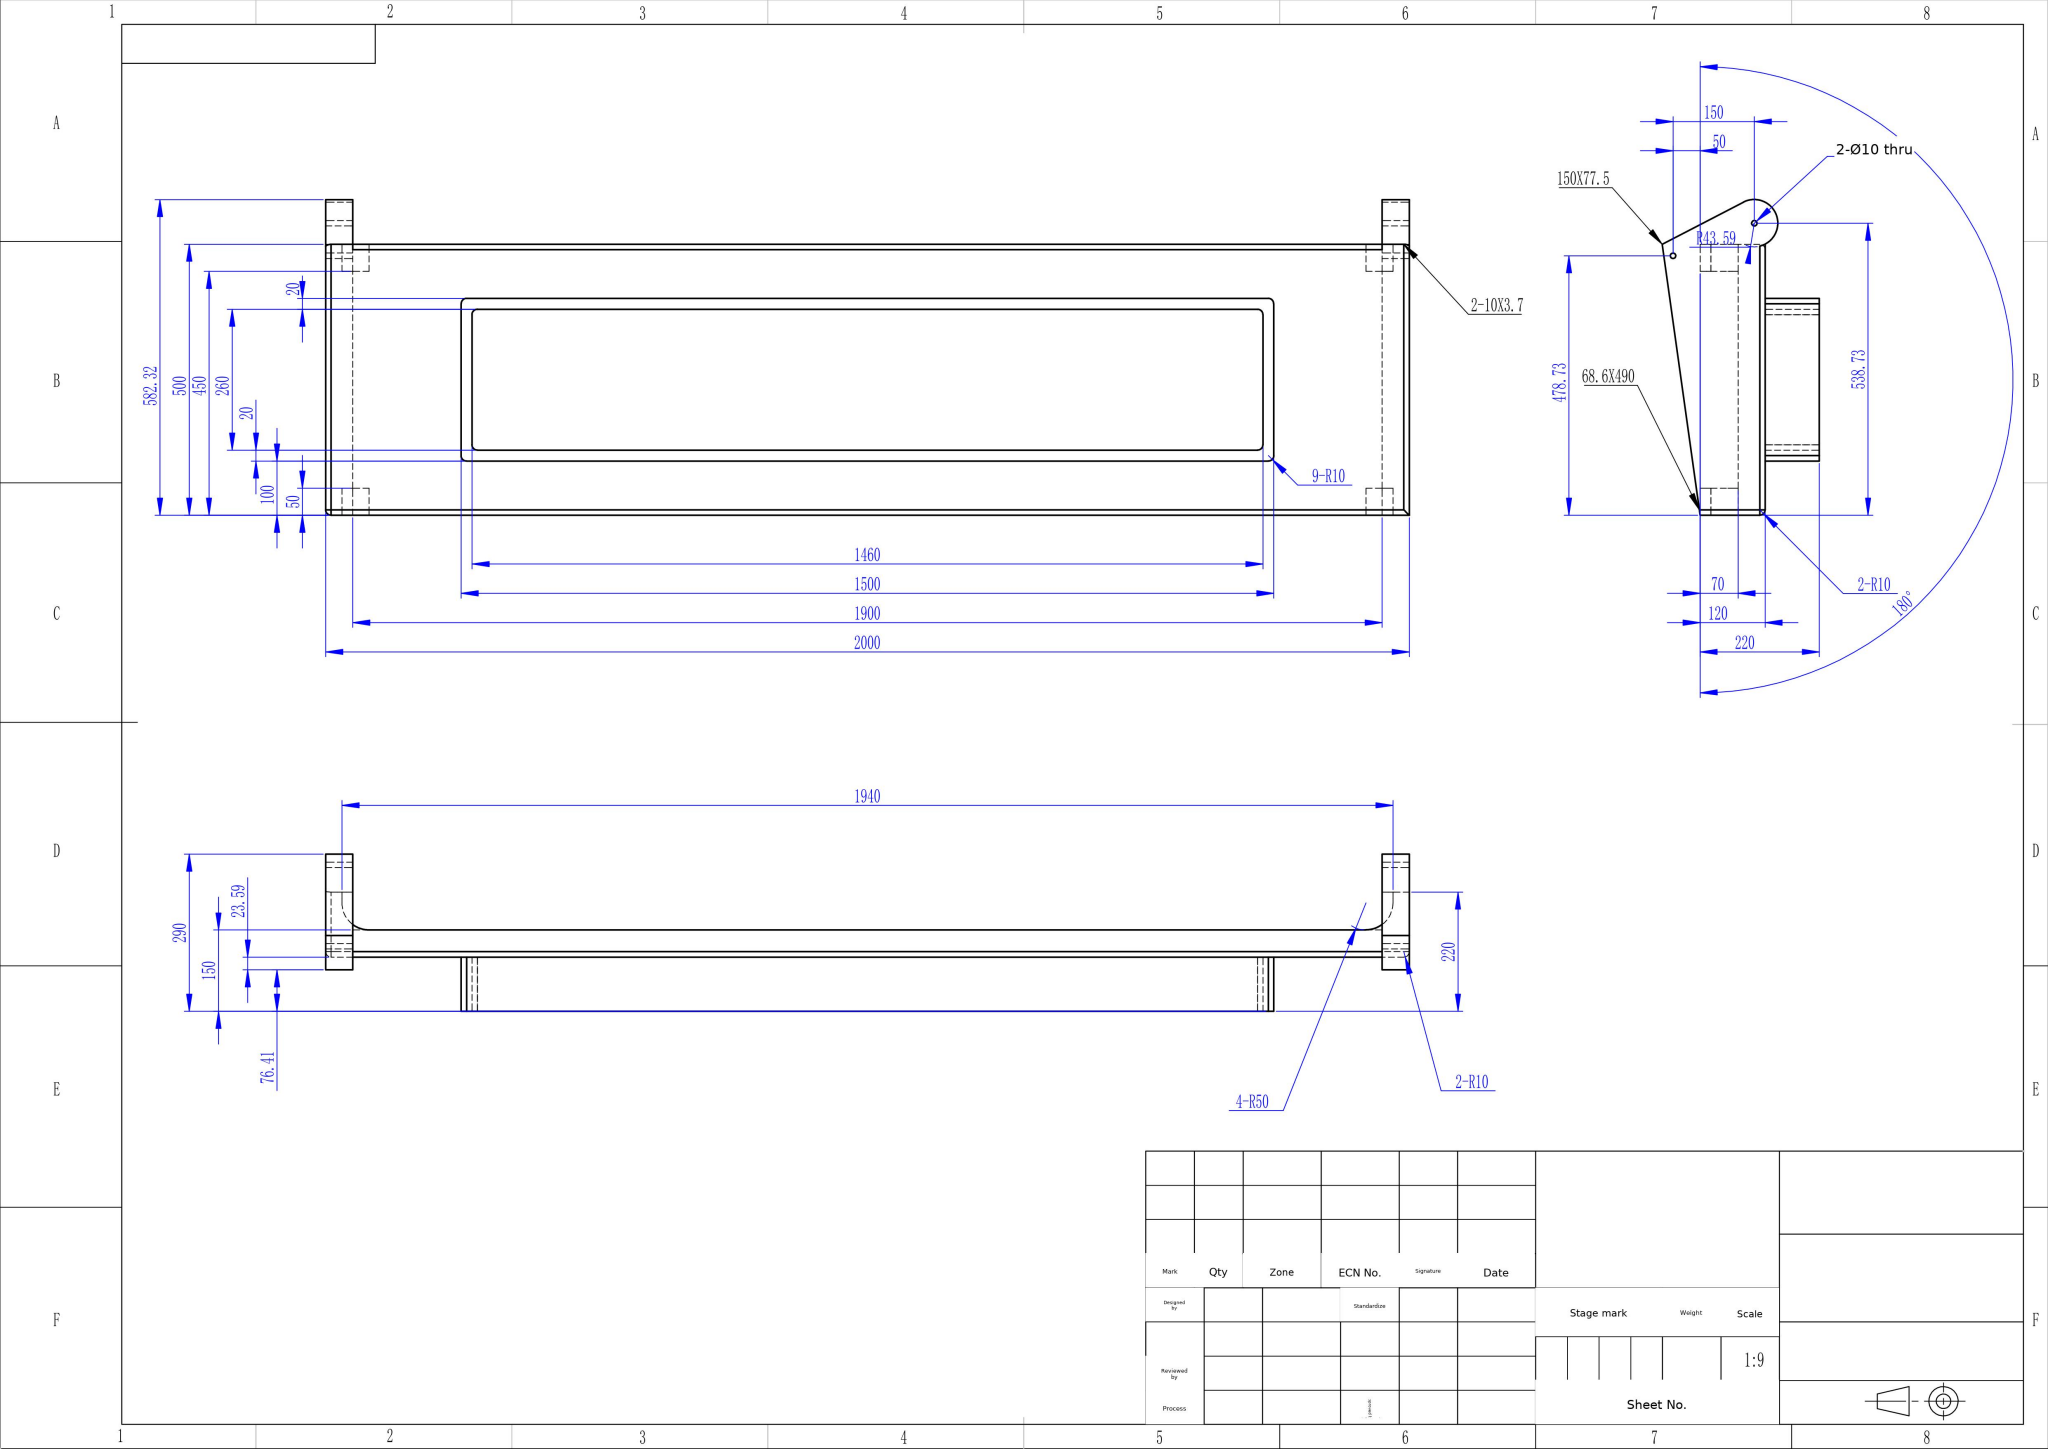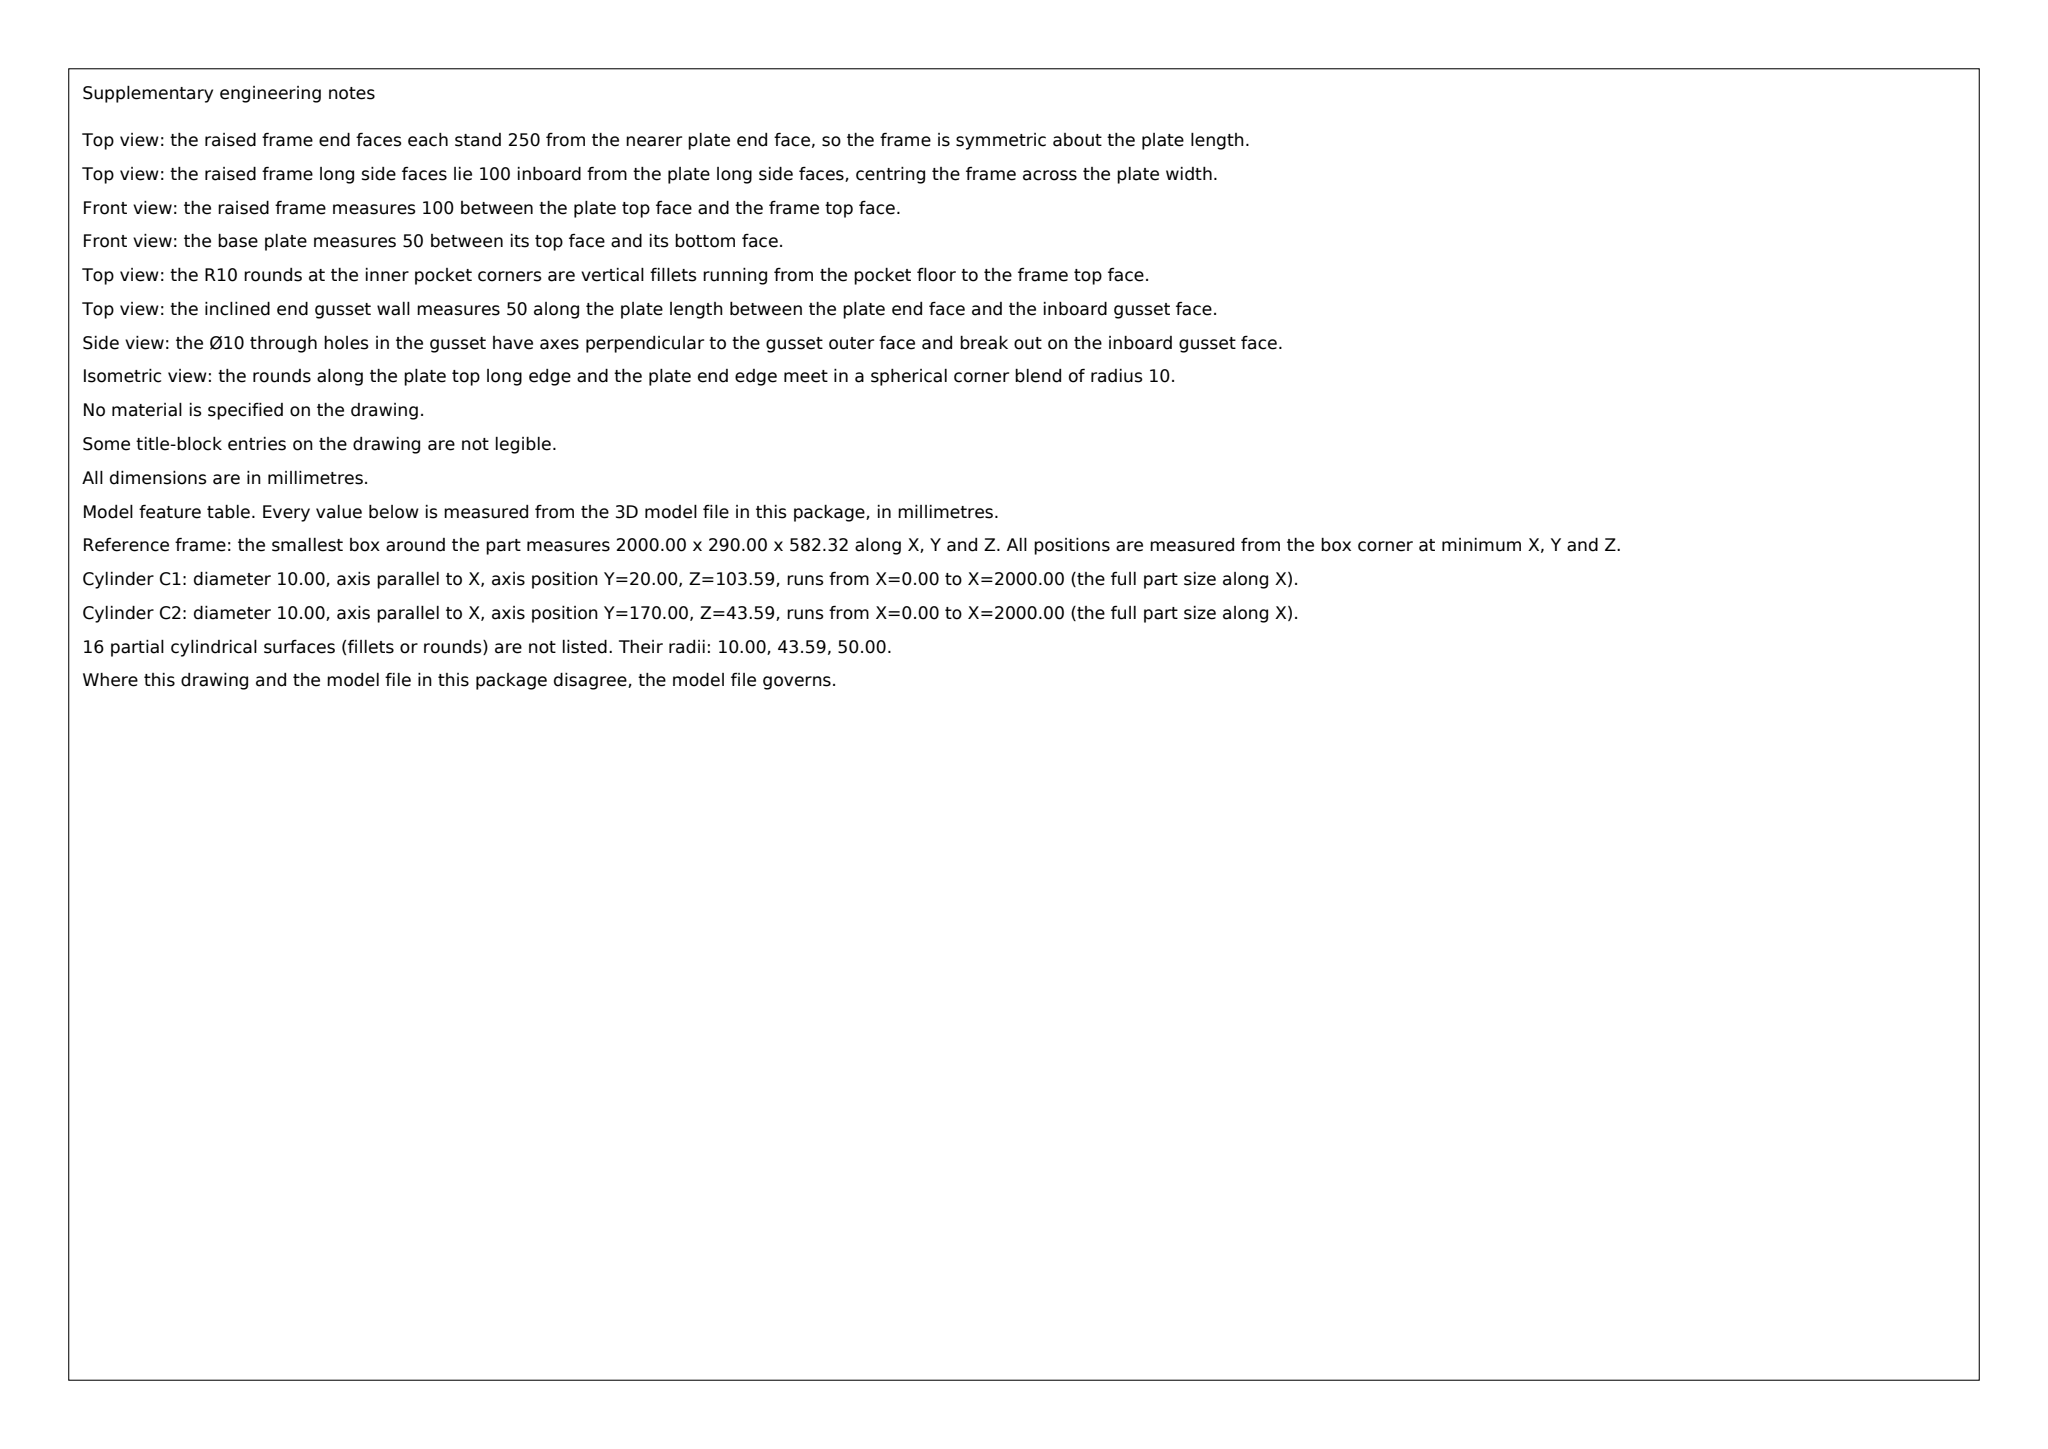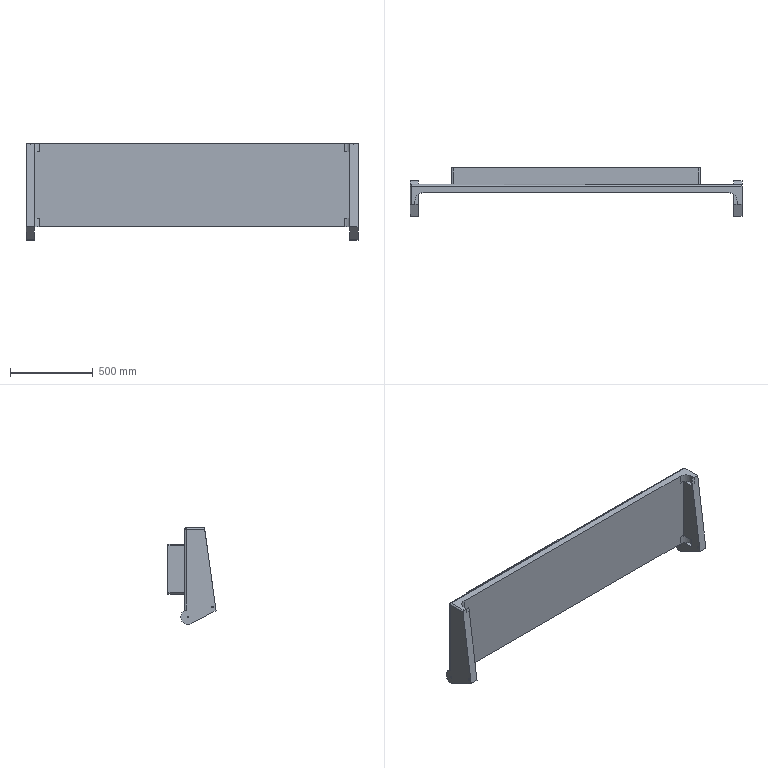Part | SolidWorks | mm | 1 solid | 69 faces | box 2000 x 290 x 582.32 mm | volume 63028481 mm3 | plane 40 | cylinder 28 | sphere 1 | commonest cylinder face diameters 20 x13 10 x8 100 x4 87.178 x3
Drawing notes:
2X Ø10 THRU END GUSSET, AXIS PARALLEL TO X, 50 DEEP FROM END FACE (X=0 AND X=2000); HOLE CENTERS AT Y=170, Z=43.59 AND Y=20, Z=103.59 FROM BBOX MIN CORNER. | from the solid: cylinders[dia,axis,pos,length]: [10.0,"x",[null,170.0,43.59],50.0] and [10.0,"x",[null,20.0,103.59],50.0]
GUSSET PLATE THICKNESS 50 ALONG X, FACES AT X=0/X=50 AND X=1950/X=2000 (SETS Ø10 HOLE AXIAL EXTENT). | from the solid: axis_planes[normal_axis,offset]: x=0.0, x=50.0, x=1950.0, x=2000.0
R43.59 ROUND END OF GUSSET IS CONCENTRIC WITH THE Ø10 HOLE AT Y=170, Z=43.59. | from the solid: cylinder [87.178,"x",[null,170.0,43.59],50.0] coincident with Ø10 hole at same y,z
ALL DIMENSIONS IN MILLIMETERS; OVERALL ENVELOPE 2000 X 290 X 582.32. | from the solid: bbox_xyz [2000.0, 290.0, 582.319] (mm)
build123d program:
from build123d import *

# Parameters (mm, degrees)
SKETCH1_W            = 2000
SKETCH1_H            = 500
BOSS_EXTRUDE1_DEPTH  = 50
BOSS_EXTRUDE2_DEPTH  = 50
MIRROR2_COPY_1_DEPTH = 50
BOSS_EXTRUDE3_DEPTH  = 50
BOSS_EXTRUDE4_DEPTH  = 50
SKETCH6_W            = 1500
SKETCH6_H            = 300
SKETCH6_W_2          = 1460
SKETCH6_H_2          = 260
BOSS_EXTRUDE5_DEPTH  = 100
FILLET2_R            = 10
FILLET3_R            = 10
SKETCH7_R            = 5
CUT_EXTRUDE1_DEPTH   = 2033.962


with BuildPart() as part:
    # Sketch1 → Boss-Extrude1 (new body)
    with BuildSketch(Plane(origin=(0, 0, 0), x_dir=(1, 0, 0), z_dir=(0, 1, 0))):
        Rectangle(SKETCH1_W, SKETCH1_H)
    extrude(amount=BOSS_EXTRUDE1_DEPTH)

    # Sketch3 → Boss-Extrude2 (add)
    with BuildSketch(Plane.XY.offset(250)):
        with BuildLine():
            Line((-1000, 0), (-1000, -70))
            Line((-1000, -70), (-970, -70))
            Line((-970, -70), (-970, -50))
            ThreePointArc((-970, -50), (-955.355, -14.645), (-920, 0))
            Line((-920, 0), (-1000, 0))
        make_face()
    boss_extrude2 = extrude(amount=-BOSS_EXTRUDE2_DEPTH)

    # Mirror1: Boss-Extrude2 across plane
    add(boss_extrude2.mirror(Plane.XY))

    # Mirror2: Boss-Extrude2 across plane
    add(boss_extrude2.mirror(Plane.ZY))

    # Mirror2 copy 1 sketch → Mirror2 copy 1 (add)
    with BuildSketch(Plane(origin=(0, 0, -250), x_dir=(-1, 0, 0), z_dir=(0, 0, -1))):
        with BuildLine():
            Line((-1000, 0), (-1000, -70))
            Line((-1000, -70), (-970, -70))
            Line((-970, -70), (-970, -50))
            ThreePointArc((-970, -50), (-955.355, -14.645), (-920, 0))
            Line((-920, 0), (-1000, 0))
        make_face()
    extrude(amount=-MIRROR2_COPY_1_DEPTH)

    # Sketch4 → Boss-Extrude3 (add)
    with BuildSketch(Plane.ZY.offset(1000)):
        Polygon((-250, -70), (-250, -140), (250, -70), (200, -70), (200, 0), (-200, 0), (-200, -70), align=None)
    boss_extrude3 = extrude(amount=-BOSS_EXTRUDE3_DEPTH)

    # Sketch5 → Boss-Extrude4 (add)
    with BuildSketch(Plane.ZY.offset(1000)):
        with BuildLine():
            ThreePointArc((-327.46, 10), (-308.73, 68.73), (-250, 50))
            Line((-250, 50), (-250, -140))
            Line((-250, -140), (-327.46, 10))
        make_face()
    boss_extrude4 = extrude(amount=-BOSS_EXTRUDE4_DEPTH)

    # Mirror3: Boss-Extrude3, Boss-Extrude4 across plane
    add(boss_extrude3.mirror(Plane.ZY))
    add(boss_extrude4.mirror(Plane.ZY))

    # Sketch6 → Boss-Extrude5 (add)
    with BuildSketch(Plane(origin=(0, 50, 0), x_dir=(1, 0, 0), z_dir=(0, 1, 0))):
        Rectangle(SKETCH6_W, SKETCH6_H)
        Rectangle(SKETCH6_W_2, SKETCH6_H_2, mode=Mode.SUBTRACT)
    extrude(amount=BOSS_EXTRUDE5_DEPTH)

    # Fillet2
    fillet2_edges = [part.edges().sort_by_distance(p)[0] for p in [
        (750, 100, 150),
        (750, 100, -150),
        (-750, 100, -150),
        (-750, 100, 150),
        (730, 100, 130),
        (730, 100, -130),
        (-730, 100, -130),
        (-730, 100, 130),
    ]]
    fillet(fillet2_edges, radius=FILLET2_R)

    # Fillet3
    fillet3_edges = [part.edges().sort_by_distance(p)[0] for p in [
        (1000, 50, 0),
        (0, 50, -250),
        (-1000, 50, 0),
        (-1000, -10, 250),
        (0, 50, 250),
    ]]
    fillet(fillet3_edges, radius=FILLET3_R)

    # Sketch7 → Cut-Extrude1 (cut, through all)
    with BuildSketch(Plane.ZY.offset(1000)):
        with Locations((-288.73, 30)):
            Circle(SKETCH7_R)
        with Locations((-228.73, -120)):
            Circle(SKETCH7_R)
    extrude(amount=-CUT_EXTRUDE1_DEPTH, mode=Mode.SUBTRACT)


solid = part.part